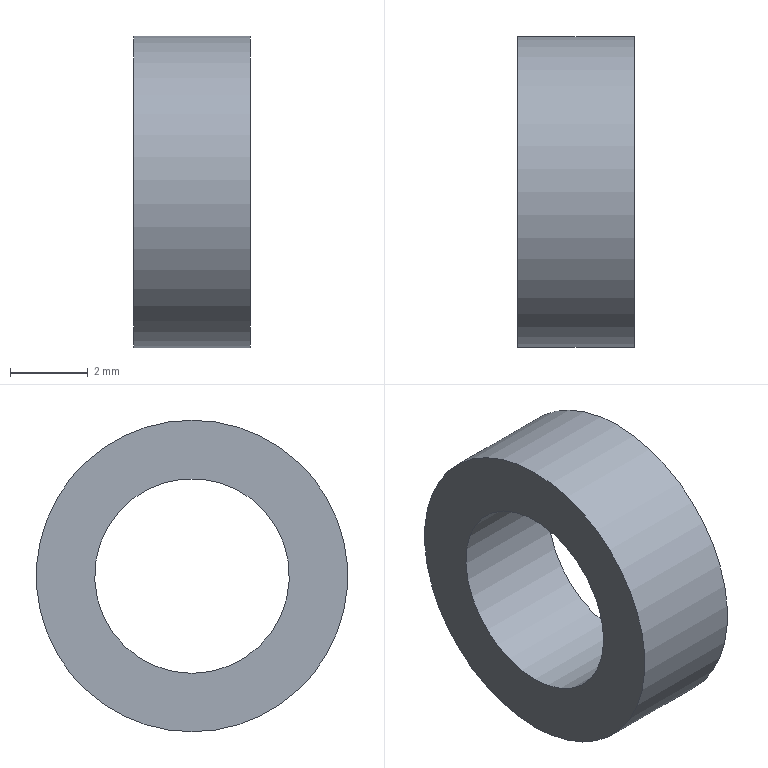Component | NX | END_CAP_3_WASHER | 1 solid | 4 faces | volume 92 mm3 | cylinder 2 | plane 2 | commonest cylinder face diameters 8 x1 5 x1